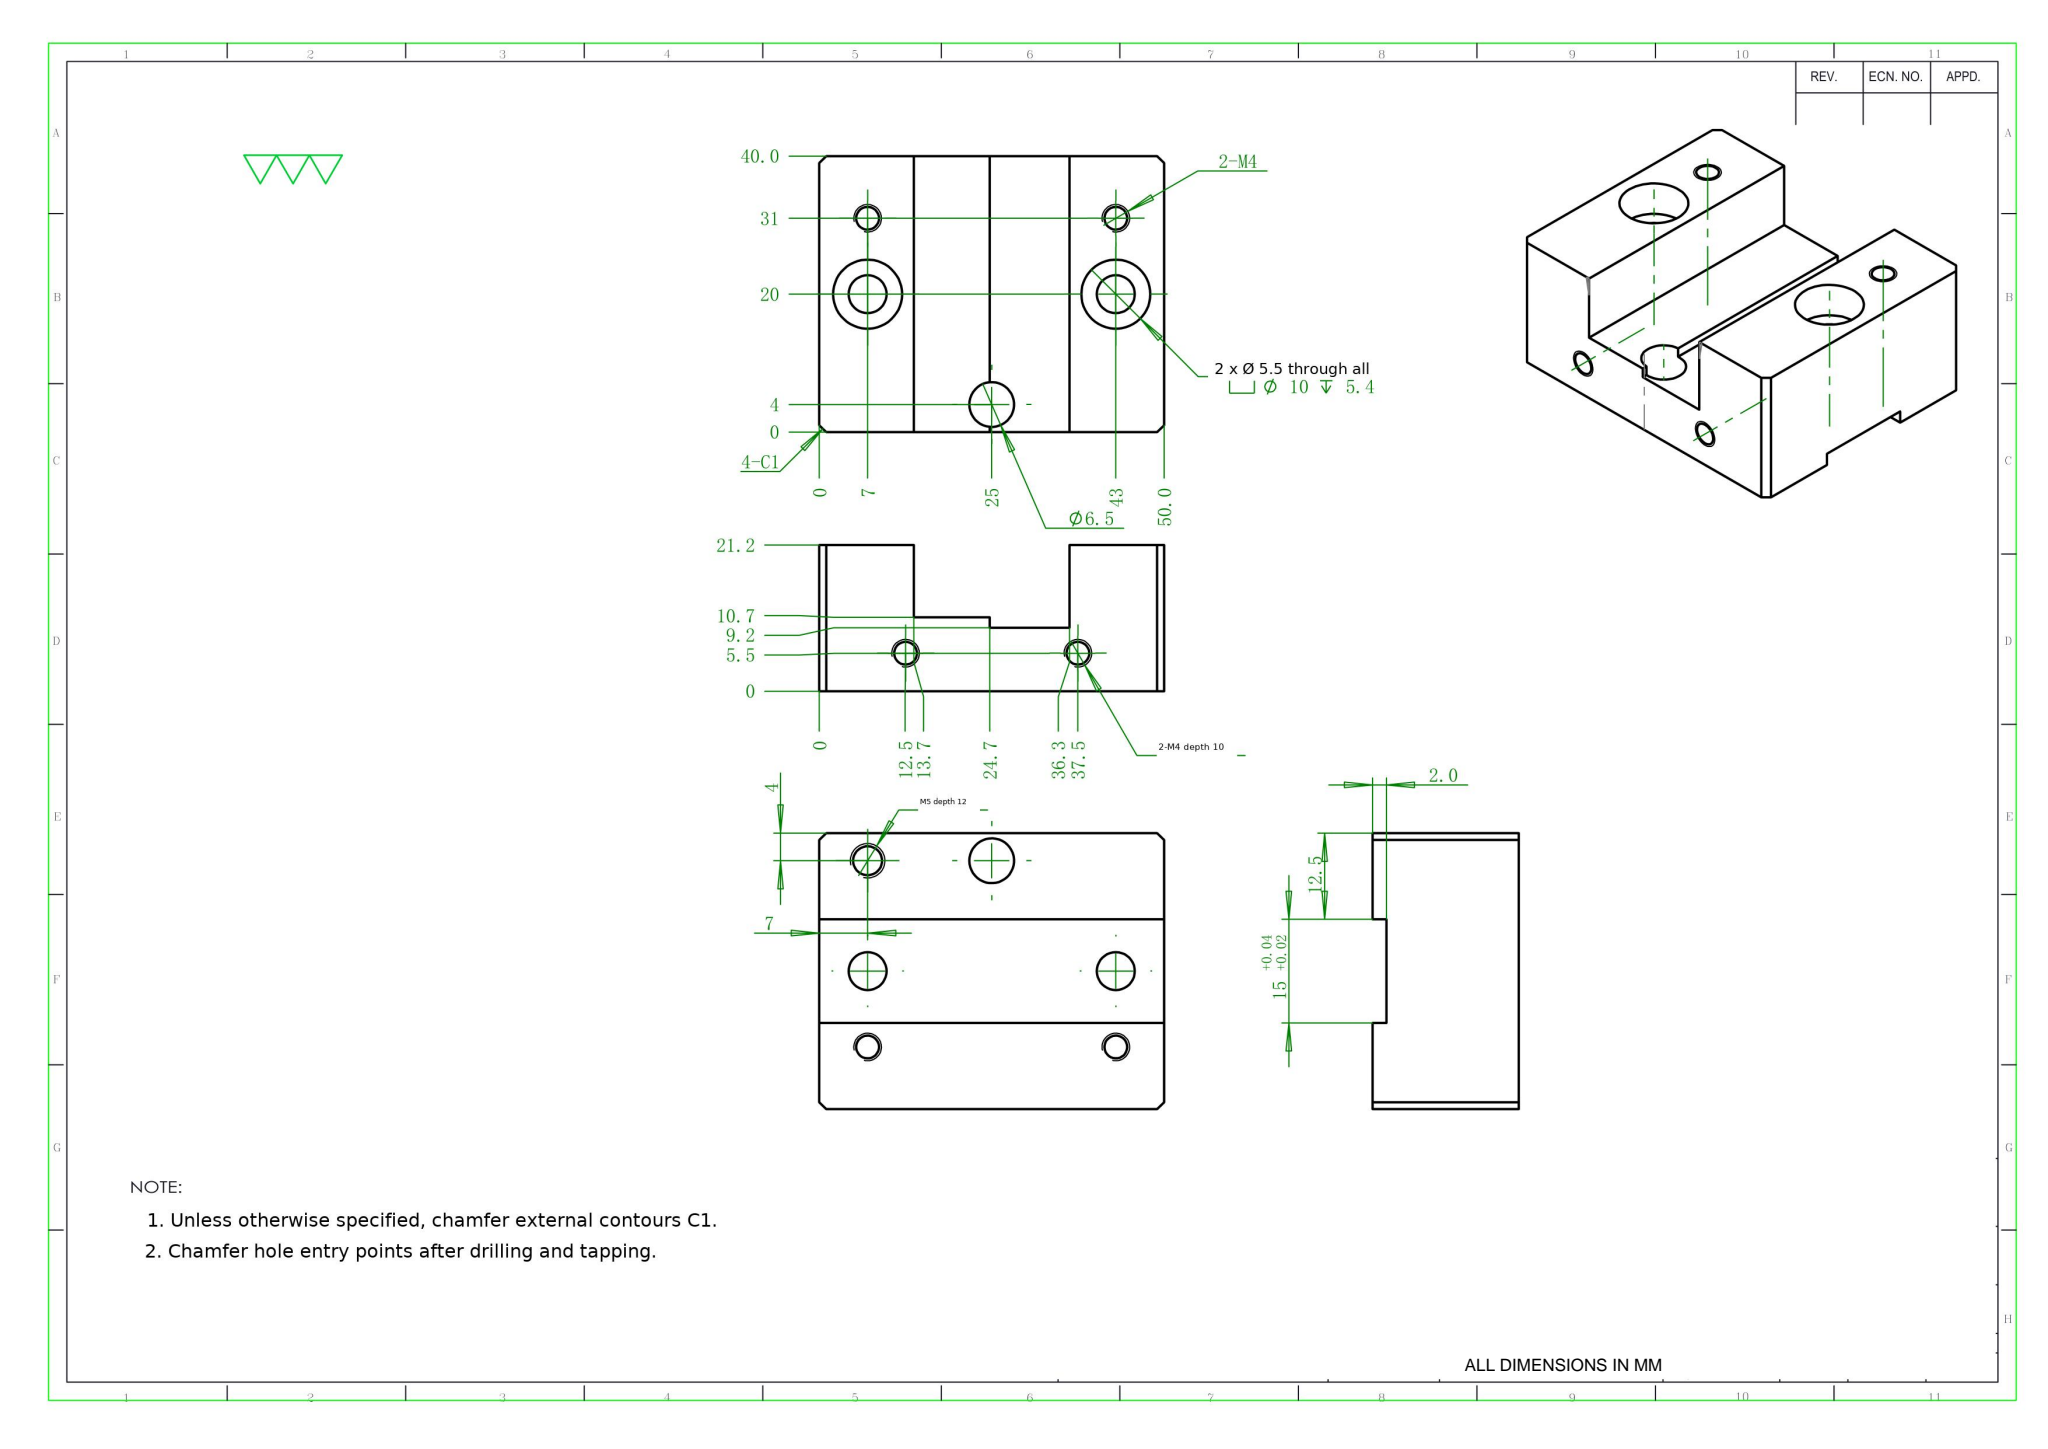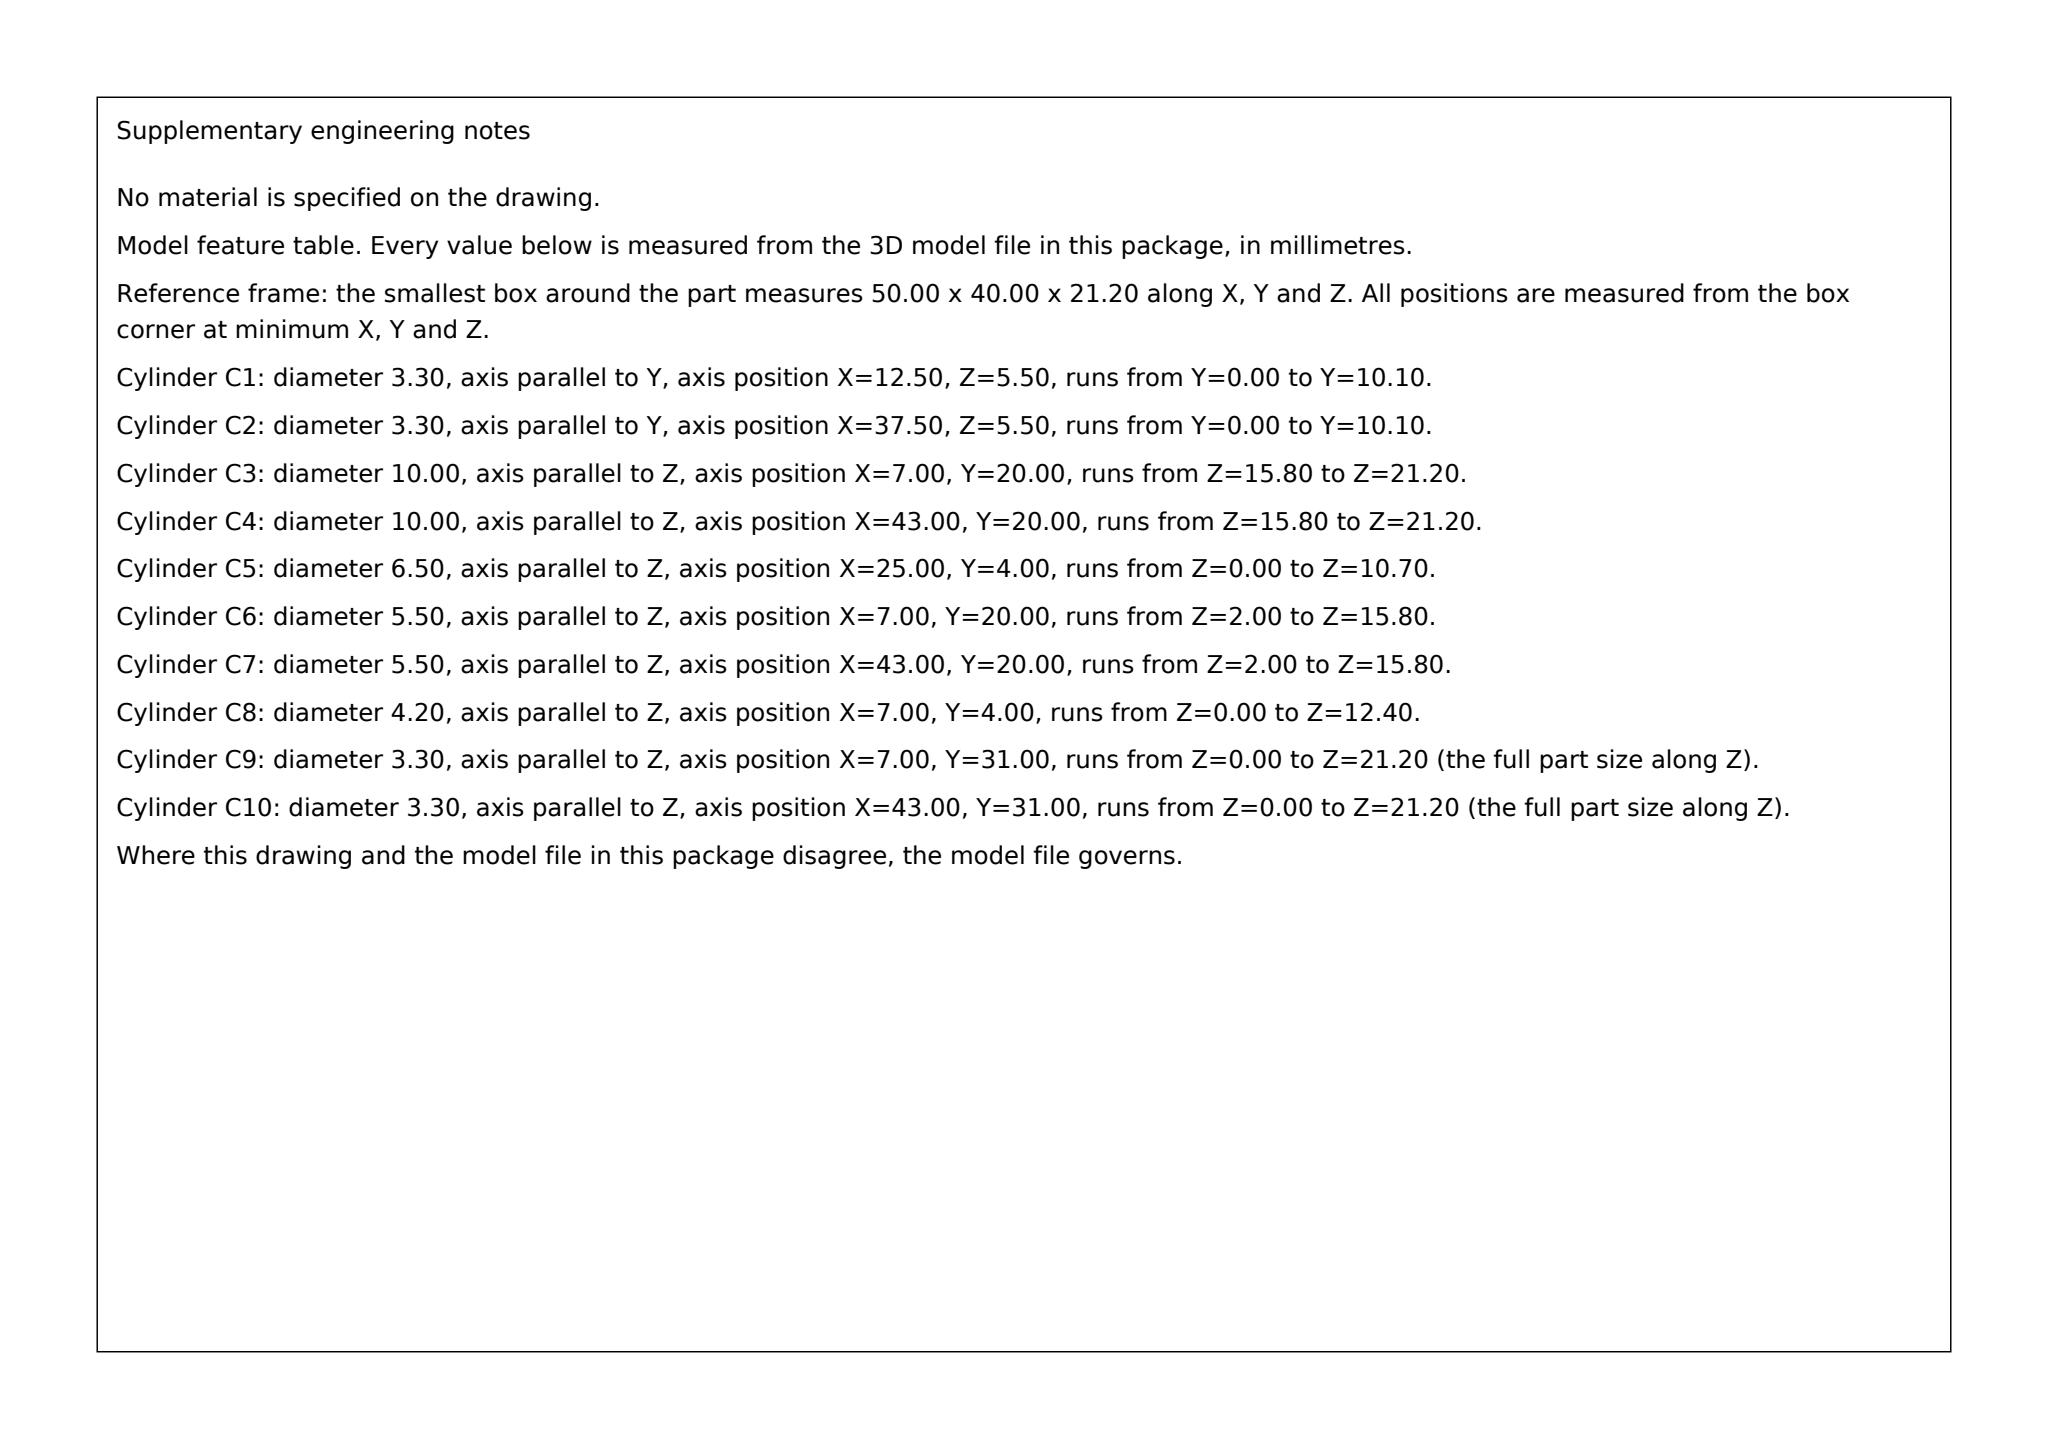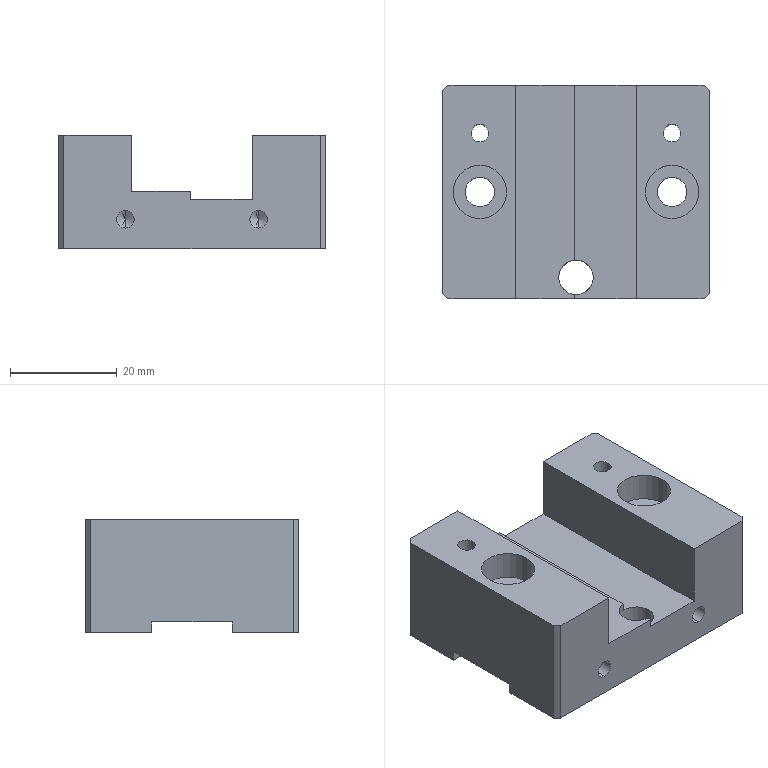Part | SolidWorks | mm | 1 solid | 49 faces | box 50 x 40 x 21.2 mm | volume 28120 mm3 | plane 23 | cylinder 20 | cone 6 | commonest cylinder face diameters 3.3 x8 10 x4 5.5 x4 4.2 x2 6.5 x2
build123d program:
from build123d import *

# Parameters (mm, degrees)
SKETCH1_W                                       = 50
SKETCH1_H                                       = 40
BOSS_EXTRUDE1_DEPTH                             = 9.2
SKETCH2_W                                       = 13.7
SKETCH2_H                                       = 40
BOSS_EXTRUDE2_DEPTH                             = 12
SKETCH17_W                                      = 11
SKETCH17_H                                      = 40
BOSS_EXTRUDE3_DEPTH                             = 1.5
M5_HEX_SOCKET_HEAD_CAP_SCREW_CBORE1_D           = 5.5
M5_HEX_SOCKET_HEAD_CAP_SCREW_CBORE1_CBORE_D     = 10
M5_HEX_SOCKET_HEAD_CAP_SCREW_CBORE1_CBORE_DEPTH = 5.4
M4_TAPPED_HOLE1_D                               = 3.3
F_6_2_6_2_DIAMETER_HOLE1_D                      = 6.5
M5_TAPPED_HOLE1_D                               = 4.2
M5_TAPPED_HOLE1_DEPTH                           = 12.4
M5_TAPPED_HOLE1_TIP                             = 1.262
M4_TAPPED_HOLE2_D                               = 3.3
M4_TAPPED_HOLE2_DEPTH                           = 10.1
M4_TAPPED_HOLE2_TIP                             = 0.9914
CHAMFER1_SIZE                                   = 1
SKETCH18_W                                      = 2
SKETCH18_H                                      = 15
CUT_EXTRUDE1_DEPTH                              = 58.874


with BuildPart() as part:
    # Sketch1 → Boss-Extrude1 (new body)
    with BuildSketch(Plane.XY):
        Rectangle(SKETCH1_W, SKETCH1_H)
    extrude(amount=BOSS_EXTRUDE1_DEPTH)

    # Sketch2 → Boss-Extrude2 (add)
    with BuildSketch(Plane.XY.offset(9.2)):
        with Locations((-18.15, 0)):
            Rectangle(SKETCH2_W, SKETCH2_H)
        with Locations((18.15, 0)):
            Rectangle(SKETCH2_W, SKETCH2_H)
    extrude(amount=BOSS_EXTRUDE2_DEPTH)

    # Sketch17 → Boss-Extrude3 (add)
    with BuildSketch(Plane.XY.offset(9.2)):
        with Locations((-5.8, 0)):
            Rectangle(SKETCH17_W, SKETCH17_H)
    extrude(amount=BOSS_EXTRUDE3_DEPTH)

    # M5 Hex Socket Head Cap Screw CBORE1 (through all)
    with Locations(Plane.XY.offset(21.2)):
        with Locations((-18, 0), (18, 0)):
            CounterBoreHole(M5_HEX_SOCKET_HEAD_CAP_SCREW_CBORE1_D / 2, M5_HEX_SOCKET_HEAD_CAP_SCREW_CBORE1_CBORE_D / 2, M5_HEX_SOCKET_HEAD_CAP_SCREW_CBORE1_CBORE_DEPTH)

    # M4 Tapped Hole1 (through all)
    with Locations(Plane.XY.offset(21.2)):
        with Locations((-18, 11), (18, 11)):
            Hole(M4_TAPPED_HOLE1_D / 2)

    # 6.2 _6.2_ Diameter Hole1 (through all)
    with Locations(Plane(origin=(0, 0, 0), x_dir=(-1, 0, 0), z_dir=(0, 0, -1))):
        with Locations((0, -16)):
            Hole(F_6_2_6_2_DIAMETER_HOLE1_D / 2)

    # M5 Tapped Hole1
    with Locations(Plane(origin=(0, 0, 0), x_dir=(-1, 0, 0), z_dir=(0, 0, -1))):
        with Locations((18, -16)):
            Hole(M5_TAPPED_HOLE1_D / 2, depth=M5_TAPPED_HOLE1_DEPTH)
            with Locations((0, 0, -(M5_TAPPED_HOLE1_DEPTH + M5_TAPPED_HOLE1_TIP / 2))):  # 118° drill point
                Cone(0, M5_TAPPED_HOLE1_D / 2, M5_TAPPED_HOLE1_TIP, mode=Mode.SUBTRACT)

    # M4 Tapped Hole2
    with Locations(Plane(origin=(0, -20, 0), x_dir=(-1, 0, 0), z_dir=(0, -1, 0))):
        with Locations((12.5, -5.5), (-12.5, -5.5)):
            Hole(M4_TAPPED_HOLE2_D / 2, depth=M4_TAPPED_HOLE2_DEPTH)
            with Locations((0, 0, -(M4_TAPPED_HOLE2_DEPTH + M4_TAPPED_HOLE2_TIP / 2))):  # 118° drill point
                Cone(0, M4_TAPPED_HOLE2_D / 2, M4_TAPPED_HOLE2_TIP, mode=Mode.SUBTRACT)

    # Chamfer1
    chamfer1_edges = [part.edges().sort_by_distance(p)[0] for p in [
        (25, -20, 10.6),
        (-25, -20, 10.6),
        (-25, 20, 10.6),
        (25, 20, 10.6),
    ]]
    chamfer(chamfer1_edges, length=CHAMFER1_SIZE)

    # Sketch18 → Cut-Extrude1 (cut, through all)
    with BuildSketch(Plane.ZY.offset(25)):
        with Locations((1, 0)):
            Rectangle(SKETCH18_W, SKETCH18_H)
    extrude(amount=-CUT_EXTRUDE1_DEPTH, mode=Mode.SUBTRACT)


solid = part.part